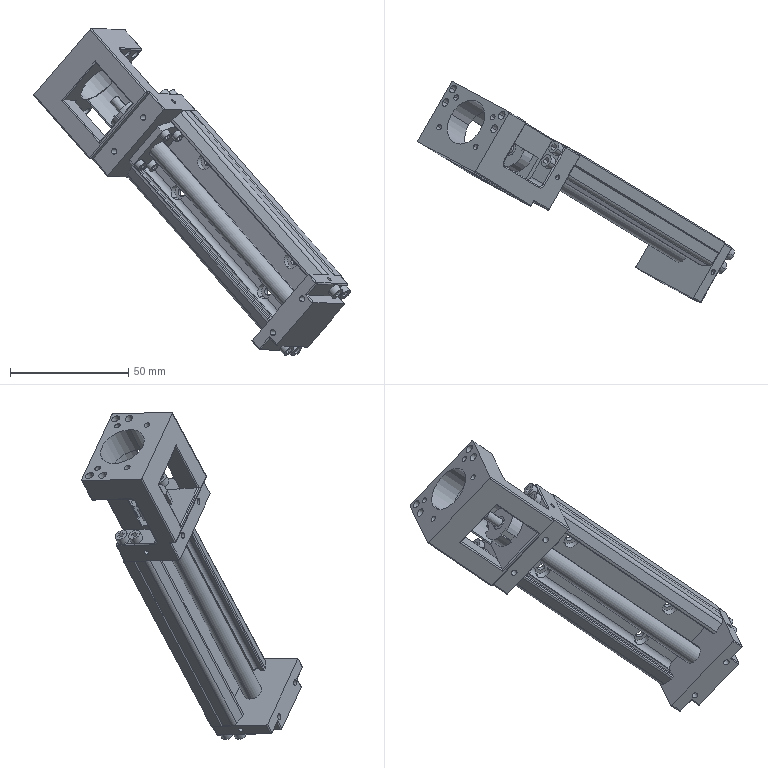Component | SolidWorks | KK40-100A1-F0z0-123-2_KK40-100_8z0-123-1 | 1 solid | 373 faces | volume 73568 mm3 | plane 196 | cylinder 163 | spline 14 | commonest cylinder face diameters 1 x41 2.5 x16 3.5 x16 5.3 x16 3 x14 6.5 x8 2.15 x8 3.4 x8